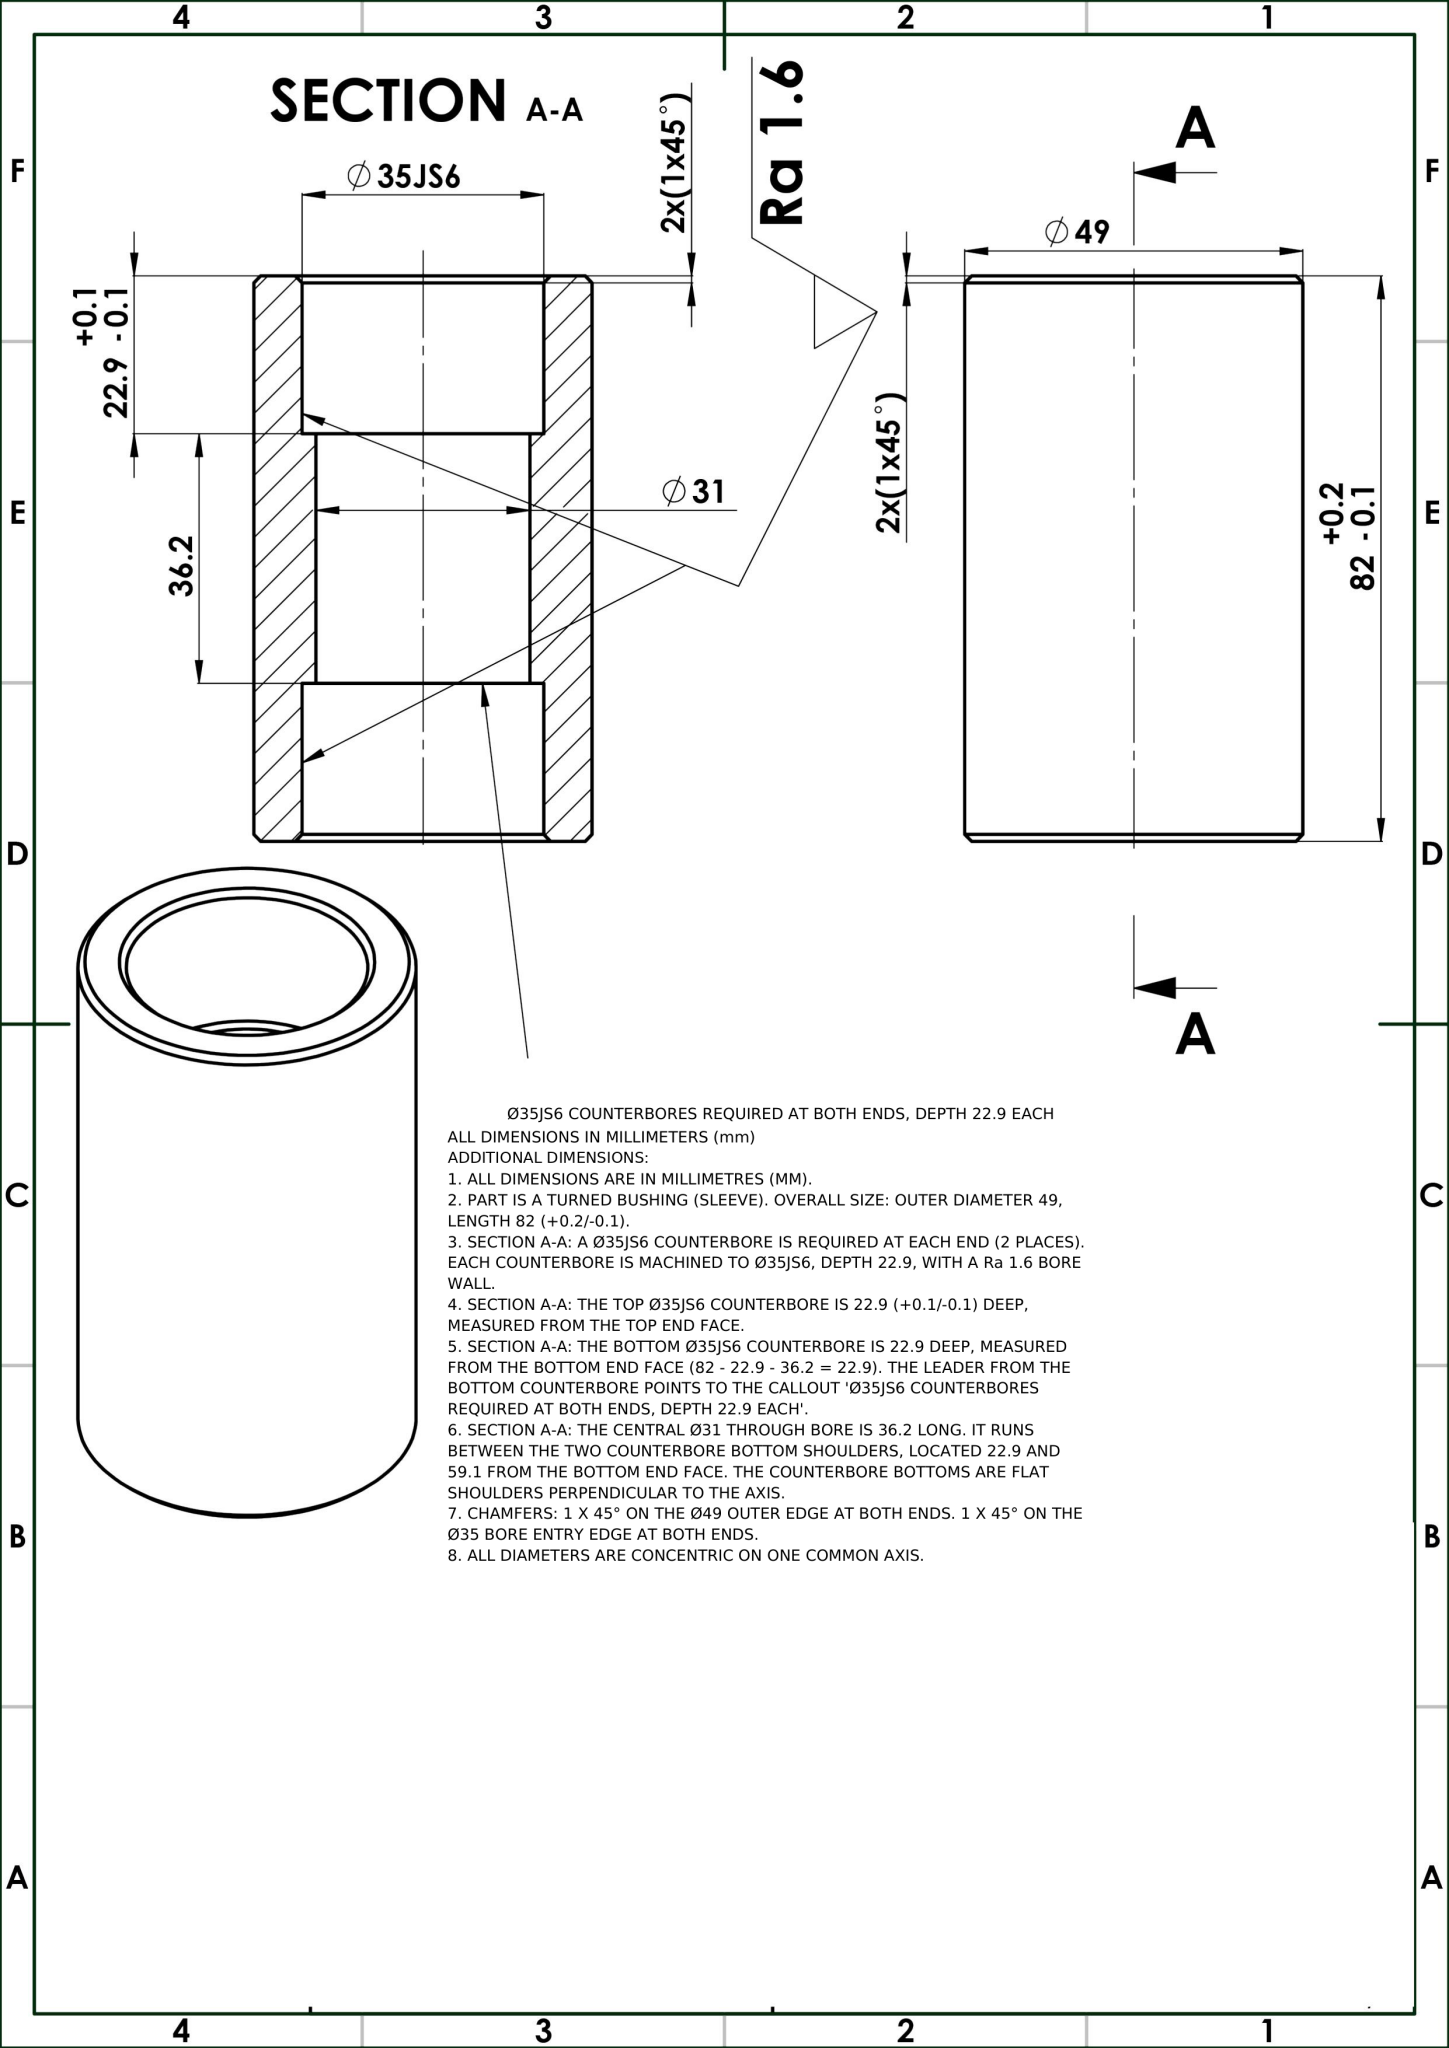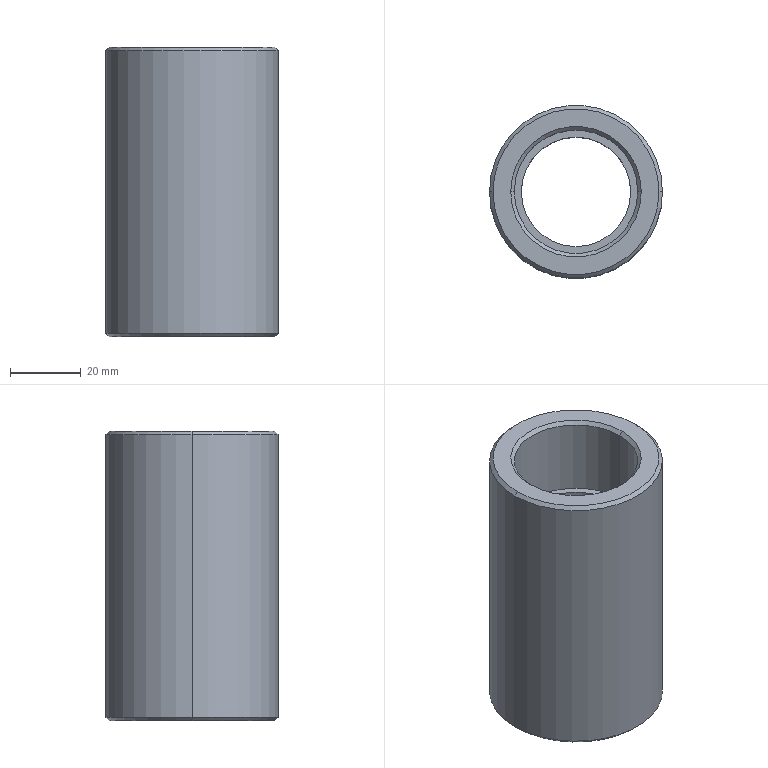Part | NX | mm | 1 solid | 20 faces | box 49 x 49 x 82 mm | volume 82980 mm3 | cone 8 | cylinder 8 | plane 4 | commonest cylinder face diameters 35 x4 31 x2 49 x2